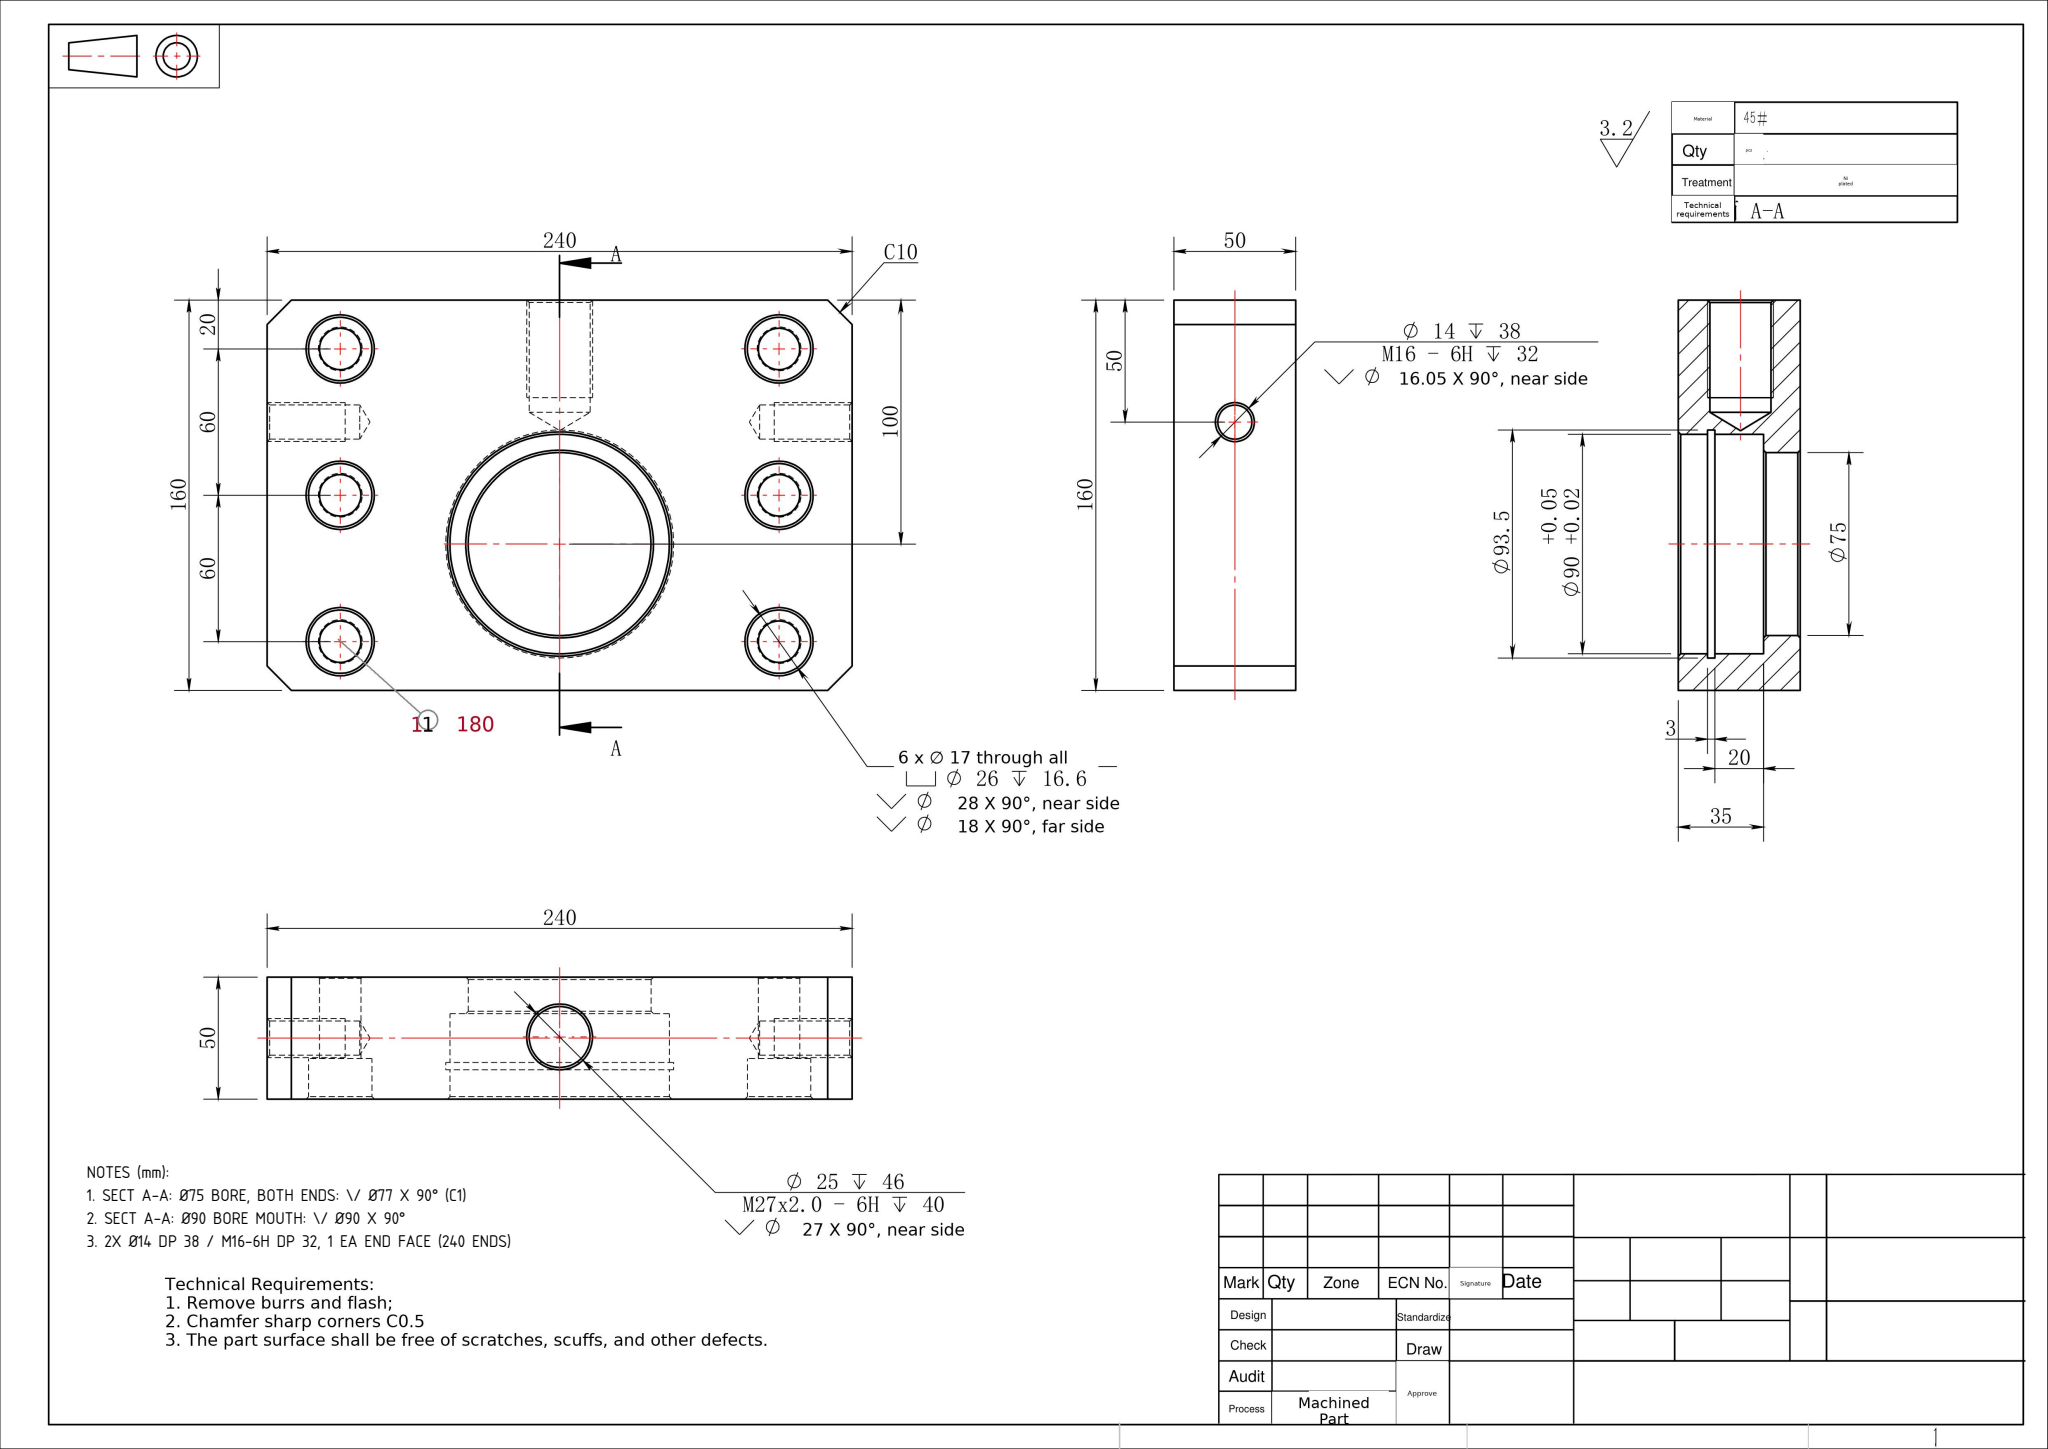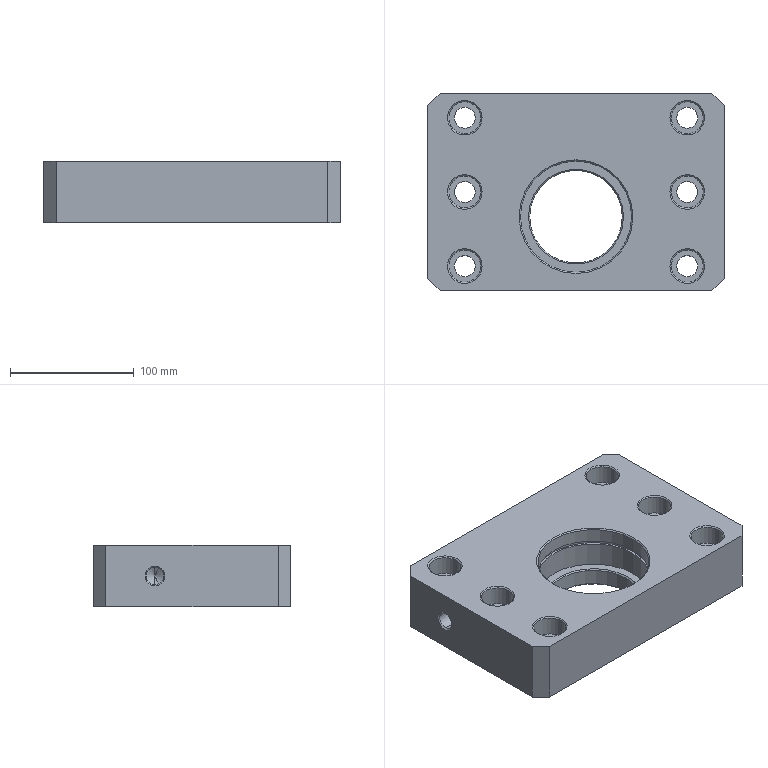Part | SolidWorks | mm | 1 solid | 99 faces | box 240 x 160 x 50 mm | volume 1484490 mm3 | cone 42 | cylinder 38 | plane 19 | commonest cylinder face diameters 26 x12 17 x12 14 x4 90 x4 25 x2 93.5 x2 75 x2
Drawing notes:
SECT A-A: Ø75 BORE, BOTH ENDS: \/ Ø77 X 90° (C1) | from the solid: cones [90.0, 77.0, 4] = 2 real chamfers on Ø75 cyl (dia75, z-axis, len 13); 90° incl, ref dia 77 -> 1 mm leg
SECT A-A: Ø90 BORE MOUTH: \/ Ø90 X 90° | from the solid: cones [90.0, 90.0, 2] = 1 real chamfer at mouth of Ø90 bore (dia90, z-axis, len 20)
2X Ø14 DP 38 / M16-6H DP 32, 1 EA END FACE (240 ENDS) | from the solid: cylinders [14.0,'x',[null,110.0,25.0],36.98,4] = 2 holes on x axis, y=110, z=25, one in each x=0/x=240 face; cones [90,16.05,4] & [118,14.0,4]